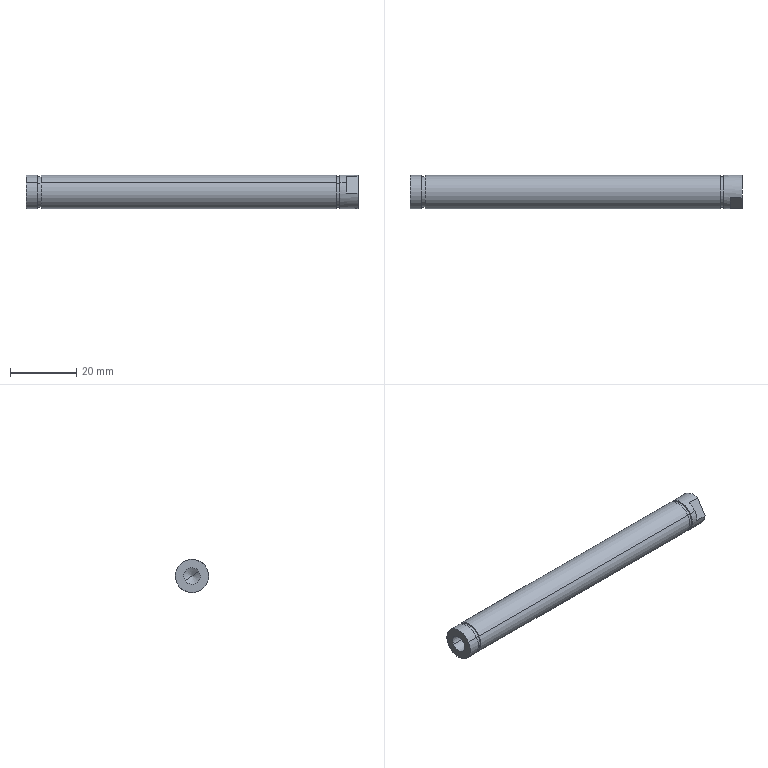Component | SolidWorks | GuideMechanism-1_SwingArm-1_GuideWheelAxis-1 | 1 solid | 24 faces | box 100 x 10 x 10 mm | volume 7573 mm3 | cylinder 12 | plane 10 | cone 2 | commonest cylinder face diameters 10 x6 9.2 x4 5 x2
build123d program:
from build123d import *

# Parameters (mm, degrees)
SKETCH1_R             = 5
BOSS_EXTRUDE1_DEPTH   = 50
CUT_EXTRUDE1_START    = -3.45
SKETCH2_R             = 5
SKETCH2_R_2           = 4.6
CUT_EXTRUDE1_DEPTH    = 1.1
LPATTERN1_COUNT       = 2
LPATTERN1_PITCH       = 90
M6_TAPPED_HOLE1_D     = 5
M6_TAPPED_HOLE1_DEPTH = 11
M6_TAPPED_HOLE1_TIP   = 1.502
SKETCH5_W             = 2.452
SKETCH5_H             = 10.703
SKETCH5_W_2           = 1.077
CUT_EXTRUDE2_DEPTH    = 3.5


with BuildPart() as part:
    # Sketch1 → Boss-Extrude1 (new, symmetric)
    with BuildSketch(Plane(origin=(0, 0, 0), x_dir=(0, 0, -1), z_dir=(1, 0, 0))):
        Circle(SKETCH1_R)
    extrude(amount=BOSS_EXTRUDE1_DEPTH, both=True)

    # Sketch2 → Cut-Extrude1 (cut)
    with BuildSketch(Plane(origin=(50, 0, 0), x_dir=(0, 0, -1), z_dir=(1, 0, 0)).offset(CUT_EXTRUDE1_START)):
        Circle(SKETCH2_R)
        Circle(SKETCH2_R_2, mode=Mode.SUBTRACT)
    cut_extrude1 = extrude(amount=-CUT_EXTRUDE1_DEPTH, mode=Mode.SUBTRACT)

    # LPattern1: Cut-Extrude1 ×2
    with Locations(*[(-i * LPATTERN1_PITCH, 0, 0) for i in range(1, LPATTERN1_COUNT)]):
        add(cut_extrude1, mode=Mode.SUBTRACT)

    # M6 Tapped Hole1
    with Locations(Plane(origin=(50, 0, 0), x_dir=(0, 0, -1), z_dir=(1, 0, 0))):
        with Locations((0, 0)):
            Hole(M6_TAPPED_HOLE1_D / 2, depth=M6_TAPPED_HOLE1_DEPTH)
            with Locations((0, 0, -(M6_TAPPED_HOLE1_DEPTH + M6_TAPPED_HOLE1_TIP / 2))):  # 118° drill point
                Cone(0, M6_TAPPED_HOLE1_D / 2, M6_TAPPED_HOLE1_TIP, mode=Mode.SUBTRACT)

    # Sketch5 → Cut-Extrude2 (cut)
    with BuildSketch(Plane.ZY.offset(50)):
        with Locations((-5.226, -0.699)):
            Rectangle(SKETCH5_W, SKETCH5_H)
        with Locations((4.539, -0.699)):
            Rectangle(SKETCH5_W_2, SKETCH5_H)
    extrude(amount=-CUT_EXTRUDE2_DEPTH, mode=Mode.SUBTRACT)


solid = part.part

# Placed as in the assembly
solid = solid.moved(Location((-446.772, -981.86, 1635), (-122.861, 0, 180)))
STEP:
#1=COLOUR_RGB('',0.7922,0.8196,0.9333);
#2=FILL_AREA_STYLE_COLOUR('',#1);
#3=FILL_AREA_STYLE('',(#2));
#4=SURFACE_STYLE_FILL_AREA(#3);
#5=SURFACE_SIDE_STYLE('',(#4));
#6=SURFACE_STYLE_USAGE(.BOTH.,#5);
#7=PRESENTATION_STYLE_ASSIGNMENT((#6));
#8=CARTESIAN_POINT('',(-19.125,-38.739,64.423));
#9=VERTEX_POINT('',#8);
#10=CARTESIAN_POINT('',(-19.125,-38.573,64.317));
#11=VERTEX_POINT('',#10);
#12=CARTESIAN_POINT('',(-19.125,-38.656,64.37));
#13=DIRECTION('',(-1.,-0.,-0.));
#14=DIRECTION('',(0.,0.84,-0.5426));
#15=AXIS2_PLACEMENT_3D('',#12,#13,#14);
#16=CIRCLE('',#15,0.09843);
#17=EDGE_CURVE('',#9,#11,#16,.T.);
#18=ORIENTED_EDGE('',*,*,#17,.F.);
#19=CARTESIAN_POINT('',(-19.558,-38.739,64.423));
#20=VERTEX_POINT('',#19);
#21=CARTESIAN_POINT('',(-19.558,-38.739,64.423));
#22=DIRECTION('',(-1.,-0.,-0.));
#23=VECTOR('',#22,39.37);
#24=LINE('',#21,#23);
#25=EDGE_CURVE('',#9,#20,#24,.T.);
#26=ORIENTED_EDGE('',*,*,#25,.T.);
#27=CARTESIAN_POINT('',(-19.558,-38.573,64.317));
#28=VERTEX_POINT('',#27);
#29=CARTESIAN_POINT('',(-19.558,-38.656,64.37));
#30=DIRECTION('',(-1.,-0.,-0.));
#31=DIRECTION('',(0.,0.84,-0.5426));
#32=AXIS2_PLACEMENT_3D('',#29,#30,#31);
#33=CIRCLE('',#32,0.09843);
#34=EDGE_CURVE('',#20,#28,#33,.T.);
#35=ORIENTED_EDGE('',*,*,#34,.T.);
#36=CARTESIAN_POINT('',(-19.558,-38.573,64.317));
#37=DIRECTION('',(-1.,-0.,-0.));
#38=VECTOR('',#37,39.37);
#39=LINE('',#36,#38);
#40=EDGE_CURVE('',#11,#28,#39,.T.);
#41=ORIENTED_EDGE('',*,*,#40,.F.);
#42=EDGE_LOOP('',(#18,#26,#35,#41));
#43=FACE_OUTER_BOUND('',#42,.T.);
#44=CARTESIAN_POINT('',(-19.558,-38.656,64.37));
#45=DIRECTION('',(-1.,-0.,-0.));
#46=DIRECTION('',(0.,0.84,-0.5426));
#47=AXIS2_PLACEMENT_3D('',#44,#45,#46);
#48=CYLINDRICAL_SURFACE('',#47,0.09843);
#49=ADVANCED_FACE('',(#43),#48,.F.);
#50=CARTESIAN_POINT('',(-19.066,-38.656,64.37));
#51=VERTEX_POINT('',#50);
#52=CARTESIAN_POINT('',(-19.125,-38.573,64.317));
#53=DIRECTION('',(-0.515,0.72,-0.4651));
#54=VECTOR('',#53,39.37);
#55=LINE('',#52,#54);
#56=EDGE_CURVE('',#51,#11,#55,.T.);
#57=ORIENTED_EDGE('',*,*,#56,.F.);
#58=CARTESIAN_POINT('',(-19.125,-38.739,64.423));
#59=DIRECTION('',(-0.515,-0.72,0.4651));
#60=VECTOR('',#59,39.37);
#61=LINE('',#58,#60);
#62=EDGE_CURVE('',#51,#9,#61,.T.);
#63=ORIENTED_EDGE('',*,*,#62,.T.);
#64=ORIENTED_EDGE('',*,*,#17,.T.);
#65=EDGE_LOOP('',(#57,#63,#64));
#66=FACE_OUTER_BOUND('',#65,.T.);
#67=CARTESIAN_POINT('',(-19.125,-38.656,64.37));
#68=DIRECTION('',(-1.,-0.,-0.));
#69=DIRECTION('',(0.,0.84,-0.5426));
#70=AXIS2_PLACEMENT_3D('',#67,#68,#69);
#71=CONICAL_SURFACE('',#70,0.09843,1.03);
#72=ADVANCED_FACE('',(#66),#71,.F.);
#73=CARTESIAN_POINT('',(-15.836,-38.491,64.263));
#74=VERTEX_POINT('',#73);
#75=CARTESIAN_POINT('',(-15.836,-38.821,64.477));
#76=VERTEX_POINT('',#75);
#77=CARTESIAN_POINT('',(-15.836,-38.656,64.37));
#78=DIRECTION('',(-1.,-0.,-0.));
#79=DIRECTION('',(0.,0.84,-0.5426));
#80=AXIS2_PLACEMENT_3D('',#77,#78,#79);
#81=CIRCLE('',#80,0.1969);
#82=EDGE_CURVE('',#74,#76,#81,.T.);
#83=ORIENTED_EDGE('',*,*,#82,.F.);
#84=CARTESIAN_POINT('',(-15.759,-38.491,64.263));
#85=VERTEX_POINT('',#84);
#86=CARTESIAN_POINT('',(-19.558,-38.491,64.263));
#87=DIRECTION('',(1.,0.,0.));
#88=VECTOR('',#87,39.37);
#89=LINE('',#86,#88);
#90=EDGE_CURVE('',#74,#85,#89,.T.);
#91=ORIENTED_EDGE('',*,*,#90,.T.);
#92=CARTESIAN_POINT('',(-15.759,-38.588,64.185));
#93=VERTEX_POINT('',#92);
#94=CARTESIAN_POINT('',(-15.759,-38.656,64.37));
#95=DIRECTION('',(1.,0.,0.));
#96=DIRECTION('',(0.,-0.84,0.5426));
#97=AXIS2_PLACEMENT_3D('',#94,#95,#96);
#98=CIRCLE('',#97,0.1969);
#99=EDGE_CURVE('',#93,#85,#98,.T.);
#100=ORIENTED_EDGE('',*,*,#99,.F.);
#101=CARTESIAN_POINT('',(-15.621,-38.588,64.185));
#102=VERTEX_POINT('',#101);
#103=CARTESIAN_POINT('',(-19.558,-38.588,64.185));
#104=DIRECTION('',(1.,0.,0.));
#105=VECTOR('',#104,39.37);
#106=LINE('',#103,#105);
#107=EDGE_CURVE('',#93,#102,#106,.T.);
#108=ORIENTED_EDGE('',*,*,#107,.T.);
#109=CARTESIAN_POINT('',(-15.621,-38.852,64.356));
#110=VERTEX_POINT('',#109);
#111=CARTESIAN_POINT('',(-15.621,-38.656,64.37));
#112=DIRECTION('',(-1.,-0.,-0.));
#113=DIRECTION('',(0.,0.84,-0.5426));
#114=AXIS2_PLACEMENT_3D('',#111,#112,#113);
#115=CIRCLE('',#114,0.1969);
#116=EDGE_CURVE('',#102,#110,#115,.T.);
#117=ORIENTED_EDGE('',*,*,#116,.T.);
#118=CARTESIAN_POINT('',(-15.759,-38.852,64.356));
#119=VERTEX_POINT('',#118);
#120=CARTESIAN_POINT('',(-19.558,-38.852,64.356));
#121=DIRECTION('',(-1.,-0.,-0.));
#122=VECTOR('',#121,39.37);
#123=LINE('',#120,#122);
#124=EDGE_CURVE('',#110,#119,#123,.T.);
#125=ORIENTED_EDGE('',*,*,#124,.T.);
#126=CARTESIAN_POINT('',(-15.759,-38.821,64.477));
#127=VERTEX_POINT('',#126);
#128=CARTESIAN_POINT('',(-15.759,-38.656,64.37));
#129=DIRECTION('',(-1.,-0.,-0.));
#130=DIRECTION('',(0.,0.84,-0.5426));
#131=AXIS2_PLACEMENT_3D('',#128,#129,#130);
#132=CIRCLE('',#131,0.1969);
#133=EDGE_CURVE('',#119,#127,#132,.T.);
#134=ORIENTED_EDGE('',*,*,#133,.T.);
#135=CARTESIAN_POINT('',(-19.558,-38.821,64.477));
#136=DIRECTION('',(1.,0.,0.));
#137=VECTOR('',#136,39.37);
#138=LINE('',#135,#137);
#139=EDGE_CURVE('',#76,#127,#138,.T.);
#140=ORIENTED_EDGE('',*,*,#139,.F.);
#141=EDGE_LOOP('',(#83,#91,#100,#108,#117,#125,#134,#140));
#142=FACE_OUTER_BOUND('',#141,.T.);
#143=CARTESIAN_POINT('',(-19.558,-38.656,64.37));
#144=DIRECTION('',(1.,0.,0.));
#145=DIRECTION('',(0.,-0.84,0.5426));
#146=AXIS2_PLACEMENT_3D('',#143,#144,#145);
#147=CYLINDRICAL_SURFACE('',#146,0.1969);
#148=ADVANCED_FACE('',(#142),#147,.T.);
#149=CARTESIAN_POINT('',(-15.879,-38.504,64.272));
#150=VERTEX_POINT('',#149);
#151=CARTESIAN_POINT('',(-15.879,-38.808,64.468));
#152=VERTEX_POINT('',#151);
#153=CARTESIAN_POINT('',(-15.879,-38.656,64.37));
#154=DIRECTION('',(-1.,-0.,-0.));
#155=DIRECTION('',(0.,0.84,-0.5426));
#156=AXIS2_PLACEMENT_3D('',#153,#154,#155);
#157=CIRCLE('',#156,0.1811);
#158=EDGE_CURVE('',#150,#152,#157,.T.);
#159=ORIENTED_EDGE('',*,*,#158,.F.);
#160=CARTESIAN_POINT('',(-15.836,-38.504,64.272));
#161=VERTEX_POINT('',#160);
#162=CARTESIAN_POINT('',(-15.879,-38.504,64.272));
#163=DIRECTION('',(1.,0.,0.));
#164=VECTOR('',#163,39.37);
#165=LINE('',#162,#164);
#166=EDGE_CURVE('',#150,#161,#165,.T.);
#167=ORIENTED_EDGE('',*,*,#166,.T.);
#168=CARTESIAN_POINT('',(-15.836,-38.808,64.468));
#169=VERTEX_POINT('',#168);
#170=CARTESIAN_POINT('',(-15.836,-38.656,64.37));
#171=DIRECTION('',(-1.,-0.,-0.));
#172=DIRECTION('',(0.,0.84,-0.5426));
#173=AXIS2_PLACEMENT_3D('',#170,#171,#172);
#174=CIRCLE('',#173,0.1811);
#175=EDGE_CURVE('',#161,#169,#174,.T.);
#176=ORIENTED_EDGE('',*,*,#175,.T.);
#177=CARTESIAN_POINT('',(-15.879,-38.808,64.468));
#178=DIRECTION('',(1.,0.,0.));
#179=VECTOR('',#178,39.37);
#180=LINE('',#177,#179);
#181=EDGE_CURVE('',#152,#169,#180,.T.);
#182=ORIENTED_EDGE('',*,*,#181,.F.);
#183=EDGE_LOOP('',(#159,#167,#176,#182));
#184=FACE_OUTER_BOUND('',#183,.T.);
#185=CARTESIAN_POINT('',(-15.879,-38.656,64.37));
#186=DIRECTION('',(1.,0.,0.));
#187=DIRECTION('',(0.,-0.84,0.5426));
#188=AXIS2_PLACEMENT_3D('',#185,#186,#187);
#189=CYLINDRICAL_SURFACE('',#188,0.1811);
#190=ADVANCED_FACE('',(#184),#189,.T.);
#191=CARTESIAN_POINT('',(-19.379,-38.491,64.263));
#192=VERTEX_POINT('',#191);
#193=CARTESIAN_POINT('',(-19.379,-38.821,64.477));
#194=VERTEX_POINT('',#193);
#195=CARTESIAN_POINT('',(-19.379,-38.656,64.37));
#196=DIRECTION('',(-1.,-0.,-0.));
#197=DIRECTION('',(0.,0.84,-0.5426));
#198=AXIS2_PLACEMENT_3D('',#195,#196,#197);
#199=CIRCLE('',#198,0.1969);
#200=EDGE_CURVE('',#192,#194,#199,.T.);
#201=ORIENTED_EDGE('',*,*,#200,.F.);
#202=CARTESIAN_POINT('',(-15.879,-38.491,64.263));
#203=VERTEX_POINT('',#202);
#204=CARTESIAN_POINT('',(-19.558,-38.491,64.263));
#205=DIRECTION('',(1.,0.,0.));
#206=VECTOR('',#205,39.37);
#207=LINE('',#204,#206);
#208=EDGE_CURVE('',#192,#203,#207,.T.);
#209=ORIENTED_EDGE('',*,*,#208,.T.);
#210=CARTESIAN_POINT('',(-15.879,-38.821,64.477));
#211=VERTEX_POINT('',#210);
#212=CARTESIAN_POINT('',(-15.879,-38.656,64.37));
#213=DIRECTION('',(-1.,-0.,-0.));
#214=DIRECTION('',(0.,0.84,-0.5426));
#215=AXIS2_PLACEMENT_3D('',#212,#213,#214);
#216=CIRCLE('',#215,0.1969);
#217=EDGE_CURVE('',#203,#211,#216,.T.);
#218=ORIENTED_EDGE('',*,*,#217,.T.);
#219=CARTESIAN_POINT('',(-19.558,-38.821,64.477));
#220=DIRECTION('',(1.,0.,0.));
#221=VECTOR('',#220,39.37);
#222=LINE('',#219,#221);
#223=EDGE_CURVE('',#194,#211,#222,.T.);
#224=ORIENTED_EDGE('',*,*,#223,.F.);
#225=EDGE_LOOP('',(#201,#209,#218,#224));
#226=FACE_OUTER_BOUND('',#225,.T.);
#227=CARTESIAN_POINT('',(-19.558,-38.656,64.37));
#228=DIRECTION('',(1.,0.,0.));
#229=DIRECTION('',(0.,-0.84,0.5426));
#230=AXIS2_PLACEMENT_3D('',#227,#228,#229);
#231=CYLINDRICAL_SURFACE('',#230,0.1969);
#232=ADVANCED_FACE('',(#226),#231,.T.);
#233=CARTESIAN_POINT('',(-19.422,-38.504,64.272));
#234=VERTEX_POINT('',#233);
#235=CARTESIAN_POINT('',(-19.422,-38.808,64.468));
#236=VERTEX_POINT('',#235);
#237=CARTESIAN_POINT('',(-19.422,-38.656,64.37));
#238=DIRECTION('',(-1.,-0.,-0.));
#239=DIRECTION('',(0.,0.84,-0.5426));
#240=AXIS2_PLACEMENT_3D('',#237,#238,#239);
#241=CIRCLE('',#240,0.1811);
#242=EDGE_CURVE('',#234,#236,#241,.T.);
#243=ORIENTED_EDGE('',*,*,#242,.F.);
#244=CARTESIAN_POINT('',(-19.379,-38.504,64.272));
#245=VERTEX_POINT('',#244);
#246=CARTESIAN_POINT('',(-19.422,-38.504,64.272));
#247=DIRECTION('',(1.,0.,0.));
#248=VECTOR('',#247,39.37);
#249=LINE('',#246,#248);
#250=EDGE_CURVE('',#234,#245,#249,.T.);
#251=ORIENTED_EDGE('',*,*,#250,.T.);
#252=CARTESIAN_POINT('',(-19.379,-38.808,64.468));
#253=VERTEX_POINT('',#252);
#254=CARTESIAN_POINT('',(-19.379,-38.656,64.37));
#255=DIRECTION('',(-1.,-0.,-0.));
#256=DIRECTION('',(0.,0.84,-0.5426));
#257=AXIS2_PLACEMENT_3D('',#254,#255,#256);
#258=CIRCLE('',#257,0.1811);
#259=EDGE_CURVE('',#245,#253,#258,.T.);
#260=ORIENTED_EDGE('',*,*,#259,.T.);
#261=CARTESIAN_POINT('',(-19.422,-38.808,64.468));
#262=DIRECTION('',(1.,0.,0.));
#263=VECTOR('',#262,39.37);
#264=LINE('',#261,#263);
#265=EDGE_CURVE('',#236,#253,#264,.T.);
#266=ORIENTED_EDGE('',*,*,#265,.F.);
#267=EDGE_LOOP('',(#243,#251,#260,#266));
#268=FACE_OUTER_BOUND('',#267,.T.);
#269=CARTESIAN_POINT('',(-19.422,-38.656,64.37));
#270=DIRECTION('',(1.,0.,0.));
#271=DIRECTION('',(0.,-0.84,0.5426));
#272=AXIS2_PLACEMENT_3D('',#269,#270,#271);
#273=CYLINDRICAL_SURFACE('',#272,0.1811);
#274=ADVANCED_FACE('',(#268),#273,.T.);
#275=CARTESIAN_POINT('',(-19.558,-38.491,64.263));
#276=VERTEX_POINT('',#275);
#277=CARTESIAN_POINT('',(-19.558,-38.821,64.477));
#278=VERTEX_POINT('',#277);
#279=CARTESIAN_POINT('',(-19.558,-38.656,64.37));
#280=DIRECTION('',(-1.,-0.,-0.));
#281=DIRECTION('',(0.,0.84,-0.5426));
#282=AXIS2_PLACEMENT_3D('',#279,#280,#281);
#283=CIRCLE('',#282,0.1969);
#284=EDGE_CURVE('',#276,#278,#283,.T.);
#285=ORIENTED_EDGE('',*,*,#284,.F.);
#286=CARTESIAN_POINT('',(-19.422,-38.491,64.263));
#287=VERTEX_POINT('',#286);
#288=CARTESIAN_POINT('',(-19.558,-38.491,64.263));
#289=DIRECTION('',(1.,0.,0.));
#290=VECTOR('',#289,39.37);
#291=LINE('',#288,#290);
#292=EDGE_CURVE('',#276,#287,#291,.T.);
#293=ORIENTED_EDGE('',*,*,#292,.T.);
#294=CARTESIAN_POINT('',(-19.422,-38.821,64.477));
#295=VERTEX_POINT('',#294);
#296=CARTESIAN_POINT('',(-19.422,-38.656,64.37));
#297=DIRECTION('',(-1.,-0.,-0.));
#298=DIRECTION('',(0.,0.84,-0.5426));
#299=AXIS2_PLACEMENT_3D('',#296,#297,#298);
#300=CIRCLE('',#299,0.1969);
#301=EDGE_CURVE('',#287,#295,#300,.T.);
#302=ORIENTED_EDGE('',*,*,#301,.T.);
#303=CARTESIAN_POINT('',(-19.558,-38.821,64.477));
#304=DIRECTION('',(1.,0.,0.));
#305=VECTOR('',#304,39.37);
#306=LINE('',#303,#305);
#307=EDGE_CURVE('',#278,#295,#306,.T.);
#308=ORIENTED_EDGE('',*,*,#307,.F.);
#309=EDGE_LOOP('',(#285,#293,#302,#308));
#310=FACE_OUTER_BOUND('',#309,.T.);
#311=CARTESIAN_POINT('',(-19.558,-38.656,64.37));
#312=DIRECTION('',(1.,0.,0.));
#313=DIRECTION('',(0.,-0.84,0.5426));
#314=AXIS2_PLACEMENT_3D('',#311,#312,#313);
#315=CYLINDRICAL_SURFACE('',#314,0.1969);
#316=ADVANCED_FACE('',(#310),#315,.T.);
#317=ORIENTED_EDGE('',*,*,#292,.F.);
#318=CARTESIAN_POINT('',(-19.558,-38.656,64.37));
#319=DIRECTION('',(-1.,-0.,-0.));
#320=DIRECTION('',(0.,0.84,-0.5426));
#321=AXIS2_PLACEMENT_3D('',#318,#319,#320);
#322=CIRCLE('',#321,0.1969);
#323=EDGE_CURVE('',#278,#276,#322,.T.);
#324=ORIENTED_EDGE('',*,*,#323,.F.);
#325=ORIENTED_EDGE('',*,*,#307,.T.);
#326=CARTESIAN_POINT('',(-19.422,-38.656,64.37));
#327=DIRECTION('',(-1.,-0.,-0.));
#328=DIRECTION('',(0.,0.84,-0.5426));
#329=AXIS2_PLACEMENT_3D('',#326,#327,#328);
#330=CIRCLE('',#329,0.1969);
#331=EDGE_CURVE('',#295,#287,#330,.T.);
#332=ORIENTED_EDGE('',*,*,#331,.T.);
#333=EDGE_LOOP('',(#317,#324,#325,#332));
#334=FACE_OUTER_BOUND('',#333,.T.);
#335=CARTESIAN_POINT('',(-19.558,-38.656,64.37));
#336=DIRECTION('',(1.,0.,0.));
#337=DIRECTION('',(0.,-0.84,0.5426));
#338=AXIS2_PLACEMENT_3D('',#335,#336,#337);
#339=CYLINDRICAL_SURFACE('',#338,0.1969);
#340=ADVANCED_FACE('',(#334),#339,.T.);
#341=CARTESIAN_POINT('',(-19.558,-38.656,64.37));
#342=DIRECTION('',(-1.,-0.,-0.));
#343=DIRECTION('',(0.,0.84,-0.5426));
#344=AXIS2_PLACEMENT_3D('',#341,#342,#343);
#345=CIRCLE('',#344,0.09843);
#346=EDGE_CURVE('',#28,#20,#345,.T.);
#347=ORIENTED_EDGE('',*,*,#346,.F.);
#348=ORIENTED_EDGE('',*,*,#34,.F.);
#349=EDGE_LOOP('',(#347,#348));
#350=FACE_BOUND('',#349,.T.);
#351=ORIENTED_EDGE('',*,*,#323,.T.);
#352=ORIENTED_EDGE('',*,*,#284,.T.);
#353=EDGE_LOOP('',(#351,#352));
#354=FACE_OUTER_BOUND('',#353,.T.);
#355=CARTESIAN_POINT('',(-19.558,-38.656,64.37));
#356=DIRECTION('',(-1.,-0.,-0.));
#357=DIRECTION('',(0.,0.84,-0.5426));
#358=AXIS2_PLACEMENT_3D('',#355,#356,#357);
#359=PLANE('',#358);
#360=ADVANCED_FACE('',(#350,#354),#359,.T.);
#361=ORIENTED_EDGE('',*,*,#331,.F.);
#362=ORIENTED_EDGE('',*,*,#301,.F.);
#363=EDGE_LOOP('',(#361,#362));
#364=FACE_OUTER_BOUND('',#363,.T.);
#365=CARTESIAN_POINT('',(-19.422,-38.656,64.37));
#366=DIRECTION('',(-1.,-0.,-0.));
#367=DIRECTION('',(0.,0.84,-0.5426));
#368=AXIS2_PLACEMENT_3D('',#365,#366,#367);
#369=CIRCLE('',#368,0.1811);
#370=EDGE_CURVE('',#236,#234,#369,.T.);
#371=ORIENTED_EDGE('',*,*,#370,.T.);
#372=ORIENTED_EDGE('',*,*,#242,.T.);
#373=EDGE_LOOP('',(#371,#372));
#374=FACE_BOUND('',#373,.T.);
#375=CARTESIAN_POINT('',(-19.422,-38.656,64.37));
#376=DIRECTION('',(-1.,-0.,-0.));
#377=DIRECTION('',(0.,0.84,-0.5426));
#378=AXIS2_PLACEMENT_3D('',#375,#376,#377);
#379=PLANE('',#378);
#380=ADVANCED_FACE('',(#364,#374),#379,.F.);
#381=CARTESIAN_POINT('',(-19.379,-38.656,64.37));
#382=DIRECTION('',(-1.,-0.,-0.));
#383=DIRECTION('',(0.,0.84,-0.5426));
#384=AXIS2_PLACEMENT_3D('',#381,#382,#383);
#385=CIRCLE('',#384,0.1969);
#386=EDGE_CURVE('',#194,#192,#385,.T.);
#387=ORIENTED_EDGE('',*,*,#386,.T.);
#388=ORIENTED_EDGE('',*,*,#200,.T.);
#389=EDGE_LOOP('',(#387,#388));
#390=FACE_OUTER_BOUND('',#389,.T.);
#391=CARTESIAN_POINT('',(-19.379,-38.656,64.37));
#392=DIRECTION('',(-1.,-0.,-0.));
#393=DIRECTION('',(0.,0.84,-0.5426));
#394=AXIS2_PLACEMENT_3D('',#391,#392,#393);
#395=CIRCLE('',#394,0.1811);
#396=EDGE_CURVE('',#253,#245,#395,.T.);
#397=ORIENTED_EDGE('',*,*,#396,.F.);
#398=ORIENTED_EDGE('',*,*,#259,.F.);
#399=EDGE_LOOP('',(#397,#398));
#400=FACE_BOUND('',#399,.T.);
#401=CARTESIAN_POINT('',(-19.379,-38.656,64.37));
#402=DIRECTION('',(-1.,-0.,-0.));
#403=DIRECTION('',(0.,0.84,-0.5426));
#404=AXIS2_PLACEMENT_3D('',#401,#402,#403);
#405=PLANE('',#404);
#406=ADVANCED_FACE('',(#390,#400),#405,.T.);
#407=ORIENTED_EDGE('',*,*,#250,.F.);
#408=ORIENTED_EDGE('',*,*,#370,.F.);
#409=ORIENTED_EDGE('',*,*,#265,.T.);
#410=ORIENTED_EDGE('',*,*,#396,.T.);
#411=EDGE_LOOP('',(#407,#408,#409,#410));
#412=FACE_OUTER_BOUND('',#411,.T.);
#413=CARTESIAN_POINT('',(-19.422,-38.656,64.37));
#414=DIRECTION('',(1.,0.,0.));
#415=DIRECTION('',(0.,-0.84,0.5426));
#416=AXIS2_PLACEMENT_3D('',#413,#414,#415);
#417=CYLINDRICAL_SURFACE('',#416,0.1811);
#418=ADVANCED_FACE('',(#412),#417,.T.);
#419=ORIENTED_EDGE('',*,*,#208,.F.);
#420=ORIENTED_EDGE('',*,*,#386,.F.);
#421=ORIENTED_EDGE('',*,*,#223,.T.);
#422=CARTESIAN_POINT('',(-15.879,-38.656,64.37));
#423=DIRECTION('',(-1.,-0.,-0.));
#424=DIRECTION('',(0.,0.84,-0.5426));
#425=AXIS2_PLACEMENT_3D('',#422,#423,#424);
#426=CIRCLE('',#425,0.1969);
#427=EDGE_CURVE('',#211,#203,#426,.T.);
#428=ORIENTED_EDGE('',*,*,#427,.T.);
#429=EDGE_LOOP('',(#419,#420,#421,#428));
#430=FACE_OUTER_BOUND('',#429,.T.);
#431=CARTESIAN_POINT('',(-19.558,-38.656,64.37));
#432=DIRECTION('',(1.,0.,0.));
#433=DIRECTION('',(0.,-0.84,0.5426));
#434=AXIS2_PLACEMENT_3D('',#431,#432,#433);
#435=CYLINDRICAL_SURFACE('',#434,0.1969);
#436=ADVANCED_FACE('',(#430),#435,.T.);
#437=ORIENTED_EDGE('',*,*,#427,.F.);
#438=ORIENTED_EDGE('',*,*,#217,.F.);
#439=EDGE_LOOP('',(#437,#438));
#440=FACE_OUTER_BOUND('',#439,.T.);
#441=CARTESIAN_POINT('',(-15.879,-38.656,64.37));
#442=DIRECTION('',(-1.,-0.,-0.));
#443=DIRECTION('',(0.,0.84,-0.5426));
#444=AXIS2_PLACEMENT_3D('',#441,#442,#443);
#445=CIRCLE('',#444,0.1811);
#446=EDGE_CURVE('',#152,#150,#445,.T.);
#447=ORIENTED_EDGE('',*,*,#446,.T.);
#448=ORIENTED_EDGE('',*,*,#158,.T.);
#449=EDGE_LOOP('',(#447,#448));
#450=FACE_BOUND('',#449,.T.);
#451=CARTESIAN_POINT('',(-15.879,-38.656,64.37));
#452=DIRECTION('',(-1.,-0.,-0.));
#453=DIRECTION('',(0.,0.84,-0.5426));
#454=AXIS2_PLACEMENT_3D('',#451,#452,#453);
#455=PLANE('',#454);
#456=ADVANCED_FACE('',(#440,#450),#455,.F.);
#457=CARTESIAN_POINT('',(-15.836,-38.656,64.37));
#458=DIRECTION('',(-1.,-0.,-0.));
#459=DIRECTION('',(0.,0.84,-0.5426));
#460=AXIS2_PLACEMENT_3D('',#457,#458,#459);
#461=CIRCLE('',#460,0.1969);
#462=EDGE_CURVE('',#76,#74,#461,.T.);
#463=ORIENTED_EDGE('',*,*,#462,.T.);
#464=ORIENTED_EDGE('',*,*,#82,.T.);
#465=EDGE_LOOP('',(#463,#464));
#466=FACE_OUTER_BOUND('',#465,.T.);
#467=CARTESIAN_POINT('',(-15.836,-38.656,64.37));
#468=DIRECTION('',(-1.,-0.,-0.));
#469=DIRECTION('',(0.,0.84,-0.5426));
#470=AXIS2_PLACEMENT_3D('',#467,#468,#469);
#471=CIRCLE('',#470,0.1811);
#472=EDGE_CURVE('',#169,#161,#471,.T.);
#473=ORIENTED_EDGE('',*,*,#472,.F.);
#474=ORIENTED_EDGE('',*,*,#175,.F.);
#475=EDGE_LOOP('',(#473,#474));
#476=FACE_BOUND('',#475,.T.);
#477=CARTESIAN_POINT('',(-15.836,-38.656,64.37));
#478=DIRECTION('',(-1.,-0.,-0.));
#479=DIRECTION('',(0.,0.84,-0.5426));
#480=AXIS2_PLACEMENT_3D('',#477,#478,#479);
#481=PLANE('',#480);
#482=ADVANCED_FACE('',(#466,#476),#481,.T.);
#483=ORIENTED_EDGE('',*,*,#166,.F.);
#484=ORIENTED_EDGE('',*,*,#446,.F.);
#485=ORIENTED_EDGE('',*,*,#181,.T.);
#486=ORIENTED_EDGE('',*,*,#472,.T.);
#487=EDGE_LOOP('',(#483,#484,#485,#486));
#488=FACE_OUTER_BOUND('',#487,.T.);
#489=CARTESIAN_POINT('',(-15.879,-38.656,64.37));
#490=DIRECTION('',(1.,0.,0.));
#491=DIRECTION('',(0.,-0.84,0.5426));
#492=AXIS2_PLACEMENT_3D('',#489,#490,#491);
#493=CYLINDRICAL_SURFACE('',#492,0.1811);
#494=ADVANCED_FACE('',(#488),#493,.T.);
#495=CARTESIAN_POINT('',(-15.621,-38.724,64.555));
#496=VERTEX_POINT('',#495);
#497=CARTESIAN_POINT('',(-15.621,-38.46,64.384));
#498=VERTEX_POINT('',#497);
#499=CARTESIAN_POINT('',(-15.621,-38.656,64.37));
#500=DIRECTION('',(-1.,-0.,-0.));
#501=DIRECTION('',(0.,0.84,-0.5426));
#502=AXIS2_PLACEMENT_3D('',#499,#500,#501);
#503=CIRCLE('',#502,0.1969);
#504=EDGE_CURVE('',#496,#498,#503,.T.);
#505=ORIENTED_EDGE('',*,*,#504,.F.);
#506=CARTESIAN_POINT('',(-15.621,-38.888,64.302));
#507=DIRECTION('',(-0.,0.5426,0.84));
#508=VECTOR('',#507,39.37);
#509=LINE('',#506,#508);
#510=EDGE_CURVE('',#110,#496,#509,.T.);
#511=ORIENTED_EDGE('',*,*,#510,.F.);
#512=ORIENTED_EDGE('',*,*,#116,.F.);
#513=CARTESIAN_POINT('',(-15.621,-38.623,64.131));
#514=DIRECTION('',(0.,-0.5426,-0.84));
#515=VECTOR('',#514,39.37);
#516=LINE('',#513,#515);
#517=EDGE_CURVE('',#498,#102,#516,.T.);
#518=ORIENTED_EDGE('',*,*,#517,.F.);
#519=EDGE_LOOP('',(#505,#511,#512,#518));
#520=FACE_OUTER_BOUND('',#519,.T.);
#521=CARTESIAN_POINT('',(-15.621,-38.656,64.37));
#522=DIRECTION('',(-1.,-0.,-0.));
#523=DIRECTION('',(0.,0.84,-0.5426));
#524=AXIS2_PLACEMENT_3D('',#521,#522,#523);
#525=PLANE('',#524);
#526=ADVANCED_FACE('',(#520),#525,.F.);
#527=ORIENTED_EDGE('',*,*,#90,.F.);
#528=ORIENTED_EDGE('',*,*,#462,.F.);
#529=ORIENTED_EDGE('',*,*,#139,.T.);
#530=CARTESIAN_POINT('',(-15.759,-38.724,64.555));
#531=VERTEX_POINT('',#530);
#532=CARTESIAN_POINT('',(-15.759,-38.656,64.37));
#533=DIRECTION('',(-1.,-0.,-0.));
#534=DIRECTION('',(0.,0.84,-0.5426));
#535=AXIS2_PLACEMENT_3D('',#532,#533,#534);
#536=CIRCLE('',#535,0.1969);
#537=EDGE_CURVE('',#127,#531,#536,.T.);
#538=ORIENTED_EDGE('',*,*,#537,.T.);
#539=CARTESIAN_POINT('',(-19.558,-38.724,64.555));
#540=DIRECTION('',(1.,0.,0.));
#541=VECTOR('',#540,39.37);
#542=LINE('',#539,#541);
#543=EDGE_CURVE('',#531,#496,#542,.T.);
#544=ORIENTED_EDGE('',*,*,#543,.T.);
#545=ORIENTED_EDGE('',*,*,#504,.T.);
#546=CARTESIAN_POINT('',(-15.759,-38.46,64.384));
#547=VERTEX_POINT('',#546);
#548=CARTESIAN_POINT('',(-19.558,-38.46,64.384));
#549=DIRECTION('',(-1.,-0.,-0.));
#550=VECTOR('',#549,39.37);
#551=LINE('',#548,#550);
#552=EDGE_CURVE('',#498,#547,#551,.T.);
#553=ORIENTED_EDGE('',*,*,#552,.T.);
#554=CARTESIAN_POINT('',(-15.759,-38.656,64.37));
#555=DIRECTION('',(1.,0.,0.));
#556=DIRECTION('',(0.,-0.84,0.5426));
#557=AXIS2_PLACEMENT_3D('',#554,#555,#556);
#558=CIRCLE('',#557,0.1969);
#559=EDGE_CURVE('',#85,#547,#558,.T.);
#560=ORIENTED_EDGE('',*,*,#559,.F.);
#561=EDGE_LOOP('',(#527,#528,#529,#538,#544,#545,#553,#560));
#562=FACE_OUTER_BOUND('',#561,.T.);
#563=CARTESIAN_POINT('',(-19.558,-38.656,64.37));
#564=DIRECTION('',(1.,0.,0.));
#565=DIRECTION('',(0.,-0.84,0.5426));
#566=AXIS2_PLACEMENT_3D('',#563,#564,#565);
#567=CYLINDRICAL_SURFACE('',#566,0.1969);
#568=ADVANCED_FACE('',(#562),#567,.T.);
#569=ORIENTED_EDGE('',*,*,#62,.F.);
#570=ORIENTED_EDGE('',*,*,#56,.T.);
#571=CARTESIAN_POINT('',(-19.125,-38.656,64.37));
#572=DIRECTION('',(-1.,-0.,-0.));
#573=DIRECTION('',(0.,0.84,-0.5426));
#574=AXIS2_PLACEMENT_3D('',#571,#572,#573);
#575=CIRCLE('',#574,0.09843);
#576=EDGE_CURVE('',#11,#9,#575,.T.);
#577=ORIENTED_EDGE('',*,*,#576,.T.);
#578=EDGE_LOOP('',(#569,#570,#577));
#579=FACE_OUTER_BOUND('',#578,.T.);
#580=CARTESIAN_POINT('',(-19.125,-38.656,64.37));
#581=DIRECTION('',(-1.,-0.,-0.));
#582=DIRECTION('',(0.,0.84,-0.5426));
#583=AXIS2_PLACEMENT_3D('',#580,#581,#582);
#584=CONICAL_SURFACE('',#583,0.09843,1.03);
#585=ADVANCED_FACE('',(#579),#584,.F.);
#586=ORIENTED_EDGE('',*,*,#25,.F.);
#587=ORIENTED_EDGE('',*,*,#576,.F.);
#588=ORIENTED_EDGE('',*,*,#40,.T.);
#589=ORIENTED_EDGE('',*,*,#346,.T.);
#590=EDGE_LOOP('',(#586,#587,#588,#589));
#591=FACE_OUTER_BOUND('',#590,.T.);
#592=CARTESIAN_POINT('',(-19.558,-38.656,64.37));
#593=DIRECTION('',(-1.,-0.,-0.));
#594=DIRECTION('',(0.,0.84,-0.5426));
#595=AXIS2_PLACEMENT_3D('',#592,#593,#594);
#596=CYLINDRICAL_SURFACE('',#595,0.09843);
#597=ADVANCED_FACE('',(#591),#596,.F.);
#598=CARTESIAN_POINT('',(-15.759,-38.623,64.131));
#599=DIRECTION('',(0.,-0.5426,-0.84));
#600=VECTOR('',#599,39.37);
#601=LINE('',#598,#600);
#602=EDGE_CURVE('',#547,#93,#601,.T.);
#603=ORIENTED_EDGE('',*,*,#602,.F.);
#604=ORIENTED_EDGE('',*,*,#552,.F.);
#605=ORIENTED_EDGE('',*,*,#517,.T.);
#606=ORIENTED_EDGE('',*,*,#107,.F.);
#607=EDGE_LOOP('',(#603,#604,#605,#606));
#608=FACE_OUTER_BOUND('',#607,.T.);
#609=CARTESIAN_POINT('',(-15.759,-38.623,64.131));
#610=DIRECTION('',(-0.,-0.84,0.5426));
#611=DIRECTION('',(-0.,0.5426,0.84));
#612=AXIS2_PLACEMENT_3D('',#609,#610,#611);
#613=PLANE('',#612);
#614=ADVANCED_FACE('',(#608),#613,.F.);
#615=ORIENTED_EDGE('',*,*,#99,.T.);
#616=ORIENTED_EDGE('',*,*,#559,.T.);
#617=ORIENTED_EDGE('',*,*,#602,.T.);
#618=EDGE_LOOP('',(#615,#616,#617));
#619=FACE_OUTER_BOUND('',#618,.T.);
#620=CARTESIAN_POINT('',(-15.759,-38.656,64.37));
#621=DIRECTION('',(1.,0.,0.));
#622=DIRECTION('',(-0.,-0.84,0.5426));
#623=AXIS2_PLACEMENT_3D('',#620,#621,#622);
#624=PLANE('',#623);
#625=ADVANCED_FACE('',(#619),#624,.T.);
#626=CARTESIAN_POINT('',(-15.759,-38.888,64.302));
#627=DIRECTION('',(-0.,0.5426,0.84));
#628=VECTOR('',#627,39.37);
#629=LINE('',#626,#628);
#630=EDGE_CURVE('',#119,#531,#629,.T.);
#631=ORIENTED_EDGE('',*,*,#630,.F.);
#632=ORIENTED_EDGE('',*,*,#124,.F.);
#633=ORIENTED_EDGE('',*,*,#510,.T.);
#634=ORIENTED_EDGE('',*,*,#543,.F.);
#635=EDGE_LOOP('',(#631,#632,#633,#634));
#636=FACE_OUTER_BOUND('',#635,.T.);
#637=CARTESIAN_POINT('',(-15.759,-38.888,64.302));
#638=DIRECTION('',(0.,0.84,-0.5426));
#639=DIRECTION('',(0.,-0.5426,-0.84));
#640=AXIS2_PLACEMENT_3D('',#637,#638,#639);
#641=PLANE('',#640);
#642=ADVANCED_FACE('',(#636),#641,.F.);
#643=ORIENTED_EDGE('',*,*,#630,.T.);
#644=ORIENTED_EDGE('',*,*,#537,.F.);
#645=ORIENTED_EDGE('',*,*,#133,.F.);
#646=EDGE_LOOP('',(#643,#644,#645));
#647=FACE_OUTER_BOUND('',#646,.T.);
#648=CARTESIAN_POINT('',(-15.759,-38.656,64.37));
#649=DIRECTION('',(-1.,-0.,-0.));
#650=DIRECTION('',(0.,0.84,-0.5426));
#651=AXIS2_PLACEMENT_3D('',#648,#649,#650);
#652=PLANE('',#651);
#653=ADVANCED_FACE('',(#647),#652,.F.);
#654=CLOSED_SHELL('',(#49,#72,#148,#190,#232,#274,#316,#340,#360,#380,#406,#418,#436,#456,#482,#494,#526,#568,#585,#597,#614,#625,#642,#653));
#655=MANIFOLD_SOLID_BREP('',#654);
#656=STYLED_ITEM('',(#7),#655);
#657=(LENGTH_UNIT()NAMED_UNIT(*)SI_UNIT($,.METRE.));
#658=LENGTH_MEASURE_WITH_UNIT(LENGTH_MEASURE(0.0254),#657);
#659=DIMENSIONAL_EXPONENTS(1.,0.,0.,0.,0.,0.,0.);
#660=(CONVERSION_BASED_UNIT('',#658)LENGTH_UNIT()NAMED_UNIT(#659));
#661=UNCERTAINTY_MEASURE_WITH_UNIT(LENGTH_MEASURE(0.00001),#660,'','');
#662=(NAMED_UNIT(*)PLANE_ANGLE_UNIT()SI_UNIT($,.RADIAN.));
#663=(NAMED_UNIT(*)SI_UNIT($,.STERADIAN.)SOLID_ANGLE_UNIT());
#664=(GEOMETRIC_REPRESENTATION_CONTEXT(3)GLOBAL_UNCERTAINTY_ASSIGNED_CONTEXT((#661))GLOBAL_UNIT_ASSIGNED_CONTEXT((#660,#662,#663))REPRESENTATION_CONTEXT('',''));
#665=MECHANICAL_DESIGN_GEOMETRIC_PRESENTATION_REPRESENTATION('',(#656),#664);
#666=PRESENTATION_LAYER_ASSIGNMENT('','',(#656));
#667=CARTESIAN_POINT('',(0.,0.,0.));
#668=DIRECTION('',(0.,0.,1.));
#669=DIRECTION('',(1.,0.,0.));
#670=AXIS2_PLACEMENT_3D('',#667,#668,#669);
#671=(LENGTH_UNIT()NAMED_UNIT(*)SI_UNIT($,.METRE.));
#672=LENGTH_MEASURE_WITH_UNIT(LENGTH_MEASURE(0.0254),#671);
#673=DIMENSIONAL_EXPONENTS(1.,0.,0.,0.,0.,0.,0.);
#674=(CONVERSION_BASED_UNIT('',#672)LENGTH_UNIT()NAMED_UNIT(#673));
#675=UNCERTAINTY_MEASURE_WITH_UNIT(LENGTH_MEASURE(0.00001),#674,'','');
#676=(NAMED_UNIT(*)PLANE_ANGLE_UNIT()SI_UNIT($,.RADIAN.));
#677=(NAMED_UNIT(*)SI_UNIT($,.STERADIAN.)SOLID_ANGLE_UNIT());
#678=(GEOMETRIC_REPRESENTATION_CONTEXT(3)GLOBAL_UNCERTAINTY_ASSIGNED_CONTEXT((#675))GLOBAL_UNIT_ASSIGNED_CONTEXT((#674,#676,#677))REPRESENTATION_CONTEXT('',''));
#679=ADVANCED_BREP_SHAPE_REPRESENTATION('',(#655,#670),#678);